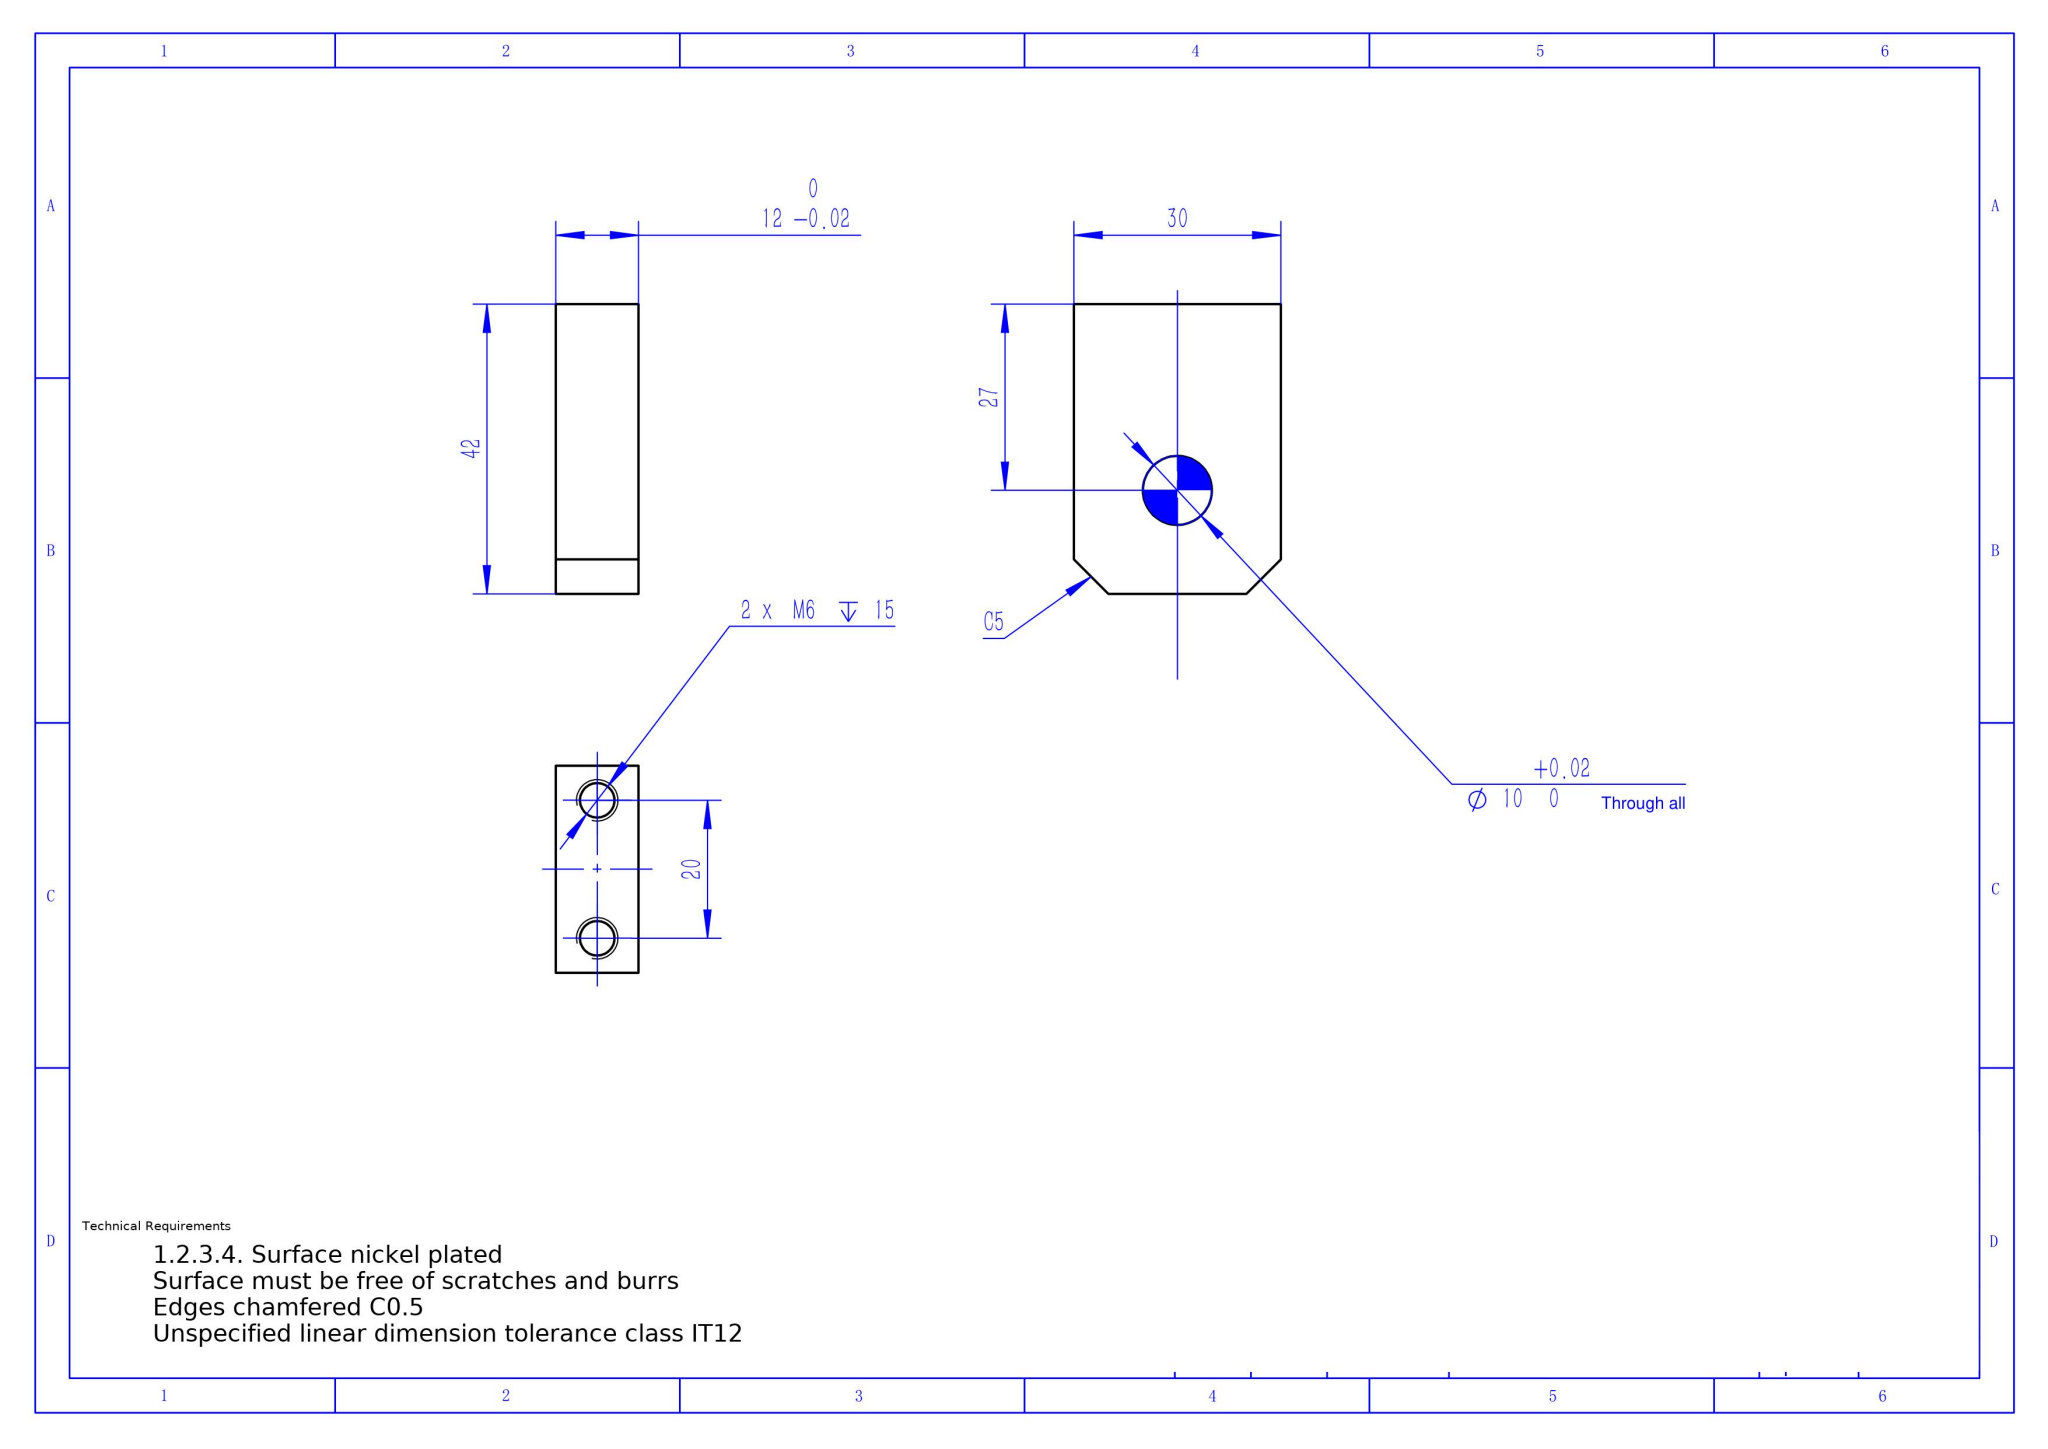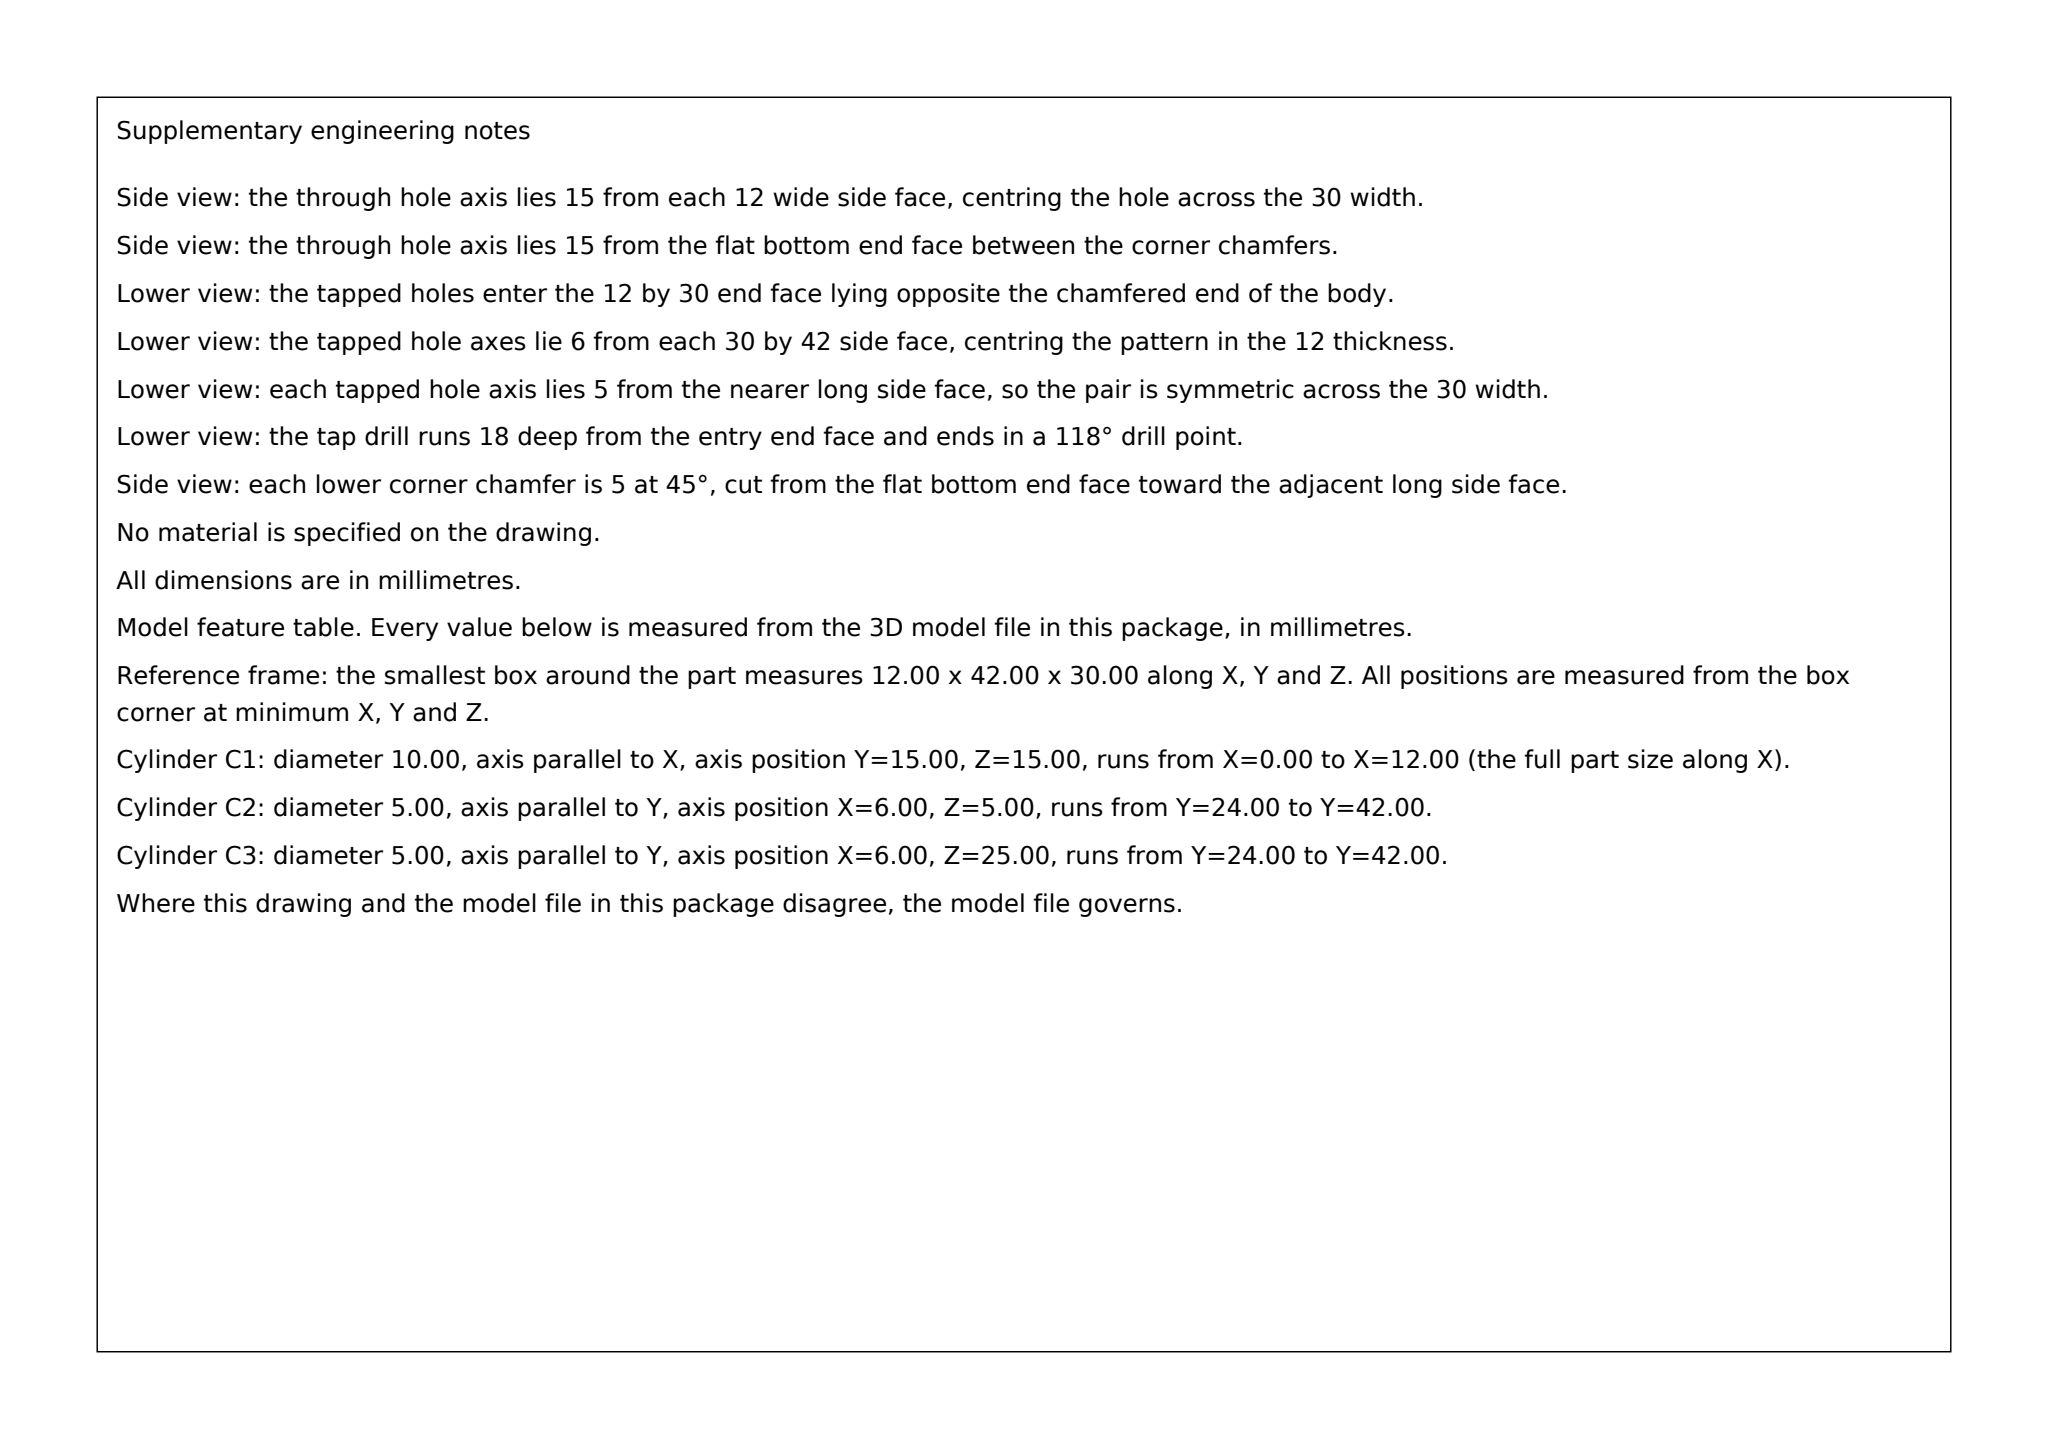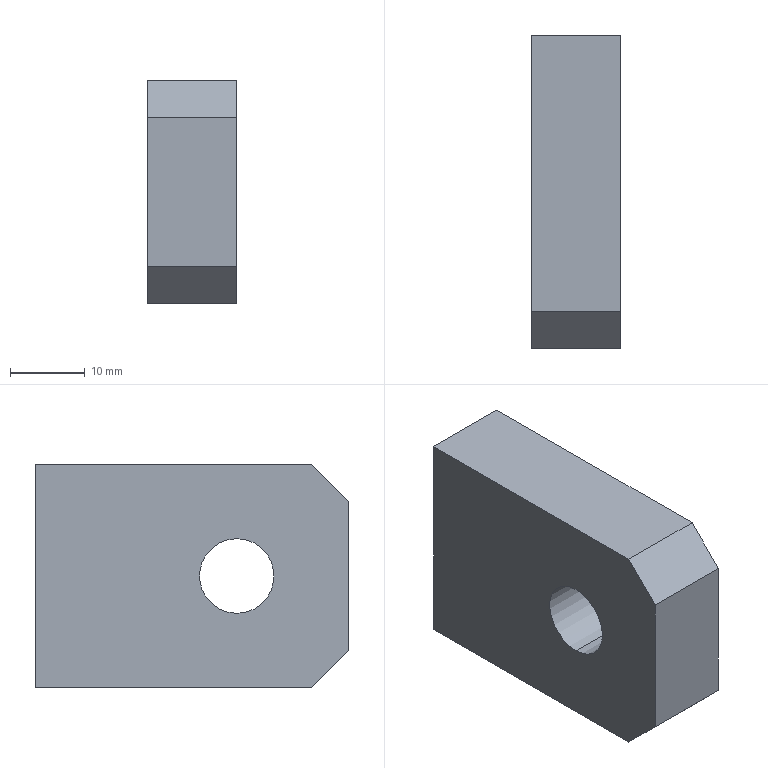Part | SolidWorks | mm | 1 solid | 18 faces | box 12 x 42 x 30 mm | volume 13151 mm3 | plane 8 | cylinder 6 | cone 4 | commonest cylinder face diameters 5 x4 10 x2
build123d program:
from build123d import *

# Parameters (mm, degrees)
SKETCH1_W                  = 30
SKETCH1_H                  = 42
BOSS_EXTRUDE1_DEPTH        = 6
SIZE_MM_DOWEL_PIN_HOLE_1_D = 10
M6_TAPPED_HOLE1_D          = 5
M6_TAPPED_HOLE1_DEPTH      = 18
M6_TAPPED_HOLE1_TIP        = 1.502
CHAMFER1_SIZE              = 5


with BuildPart() as part:
    # Sketch1 → Boss-Extrude1 (new, symmetric)
    with BuildSketch(Plane(origin=(0, 0, 0), x_dir=(0, 0, -1), z_dir=(1, 0, 0))):
        with Locations((0, 21)):
            Rectangle(SKETCH1_W, SKETCH1_H)
    extrude(amount=BOSS_EXTRUDE1_DEPTH, both=True)

    # Size mm Dowel Pin Hole 1 (through all)
    with Locations(Plane(origin=(6, 0, 0), x_dir=(0, 0, -1), z_dir=(1, 0, 0))):
        with Locations((0, 15)):
            Hole(SIZE_MM_DOWEL_PIN_HOLE_1_D / 2)

    # M6 Tapped Hole1
    with Locations(Plane(origin=(0, 42, -226.777), x_dir=(1, 0, 0), z_dir=(0, 1, 0))):
        with Locations((0, -216.777), (0, -236.777)):
            Hole(M6_TAPPED_HOLE1_D / 2, depth=M6_TAPPED_HOLE1_DEPTH)
            with Locations((0, 0, -(M6_TAPPED_HOLE1_DEPTH + M6_TAPPED_HOLE1_TIP / 2))):  # 118° drill point
                Cone(0, M6_TAPPED_HOLE1_D / 2, M6_TAPPED_HOLE1_TIP, mode=Mode.SUBTRACT)

    # Chamfer1
    chamfer1_edges = [part.edges().sort_by_distance(p)[0] for p in [
        (0, 0, -15),
        (0, 0, 15),
    ]]
    chamfer(chamfer1_edges, length=CHAMFER1_SIZE)


solid = part.part
STEP:
#1=CARTESIAN_POINT('',(0.,24.,-12.5));
#2=VERTEX_POINT('',#1);
#3=CARTESIAN_POINT('',(0.,24.,-7.5));
#4=VERTEX_POINT('',#3);
#5=CARTESIAN_POINT('',(0.,24.,-10.));
#6=DIRECTION('',(0.,1.,0.));
#7=DIRECTION('',(0.,0.,1.));
#8=AXIS2_PLACEMENT_3D('',#5,#6,#7);
#9=CIRCLE('',#8,2.5);
#10=EDGE_CURVE('',#2,#4,#9,.T.);
#11=ORIENTED_EDGE('',*,*,#10,.F.);
#12=CARTESIAN_POINT('',(0.,42.,-12.5));
#13=VERTEX_POINT('',#12);
#14=CARTESIAN_POINT('',(0.,42.,-12.5));
#15=DIRECTION('',(0.,1.,0.));
#16=VECTOR('',#15,1000.);
#17=LINE('',#14,#16);
#18=EDGE_CURVE('',#2,#13,#17,.T.);
#19=ORIENTED_EDGE('',*,*,#18,.T.);
#20=CARTESIAN_POINT('',(0.,42.,-7.5));
#21=VERTEX_POINT('',#20);
#22=CARTESIAN_POINT('',(0.,42.,-10.));
#23=DIRECTION('',(0.,1.,0.));
#24=DIRECTION('',(0.,0.,1.));
#25=AXIS2_PLACEMENT_3D('',#22,#23,#24);
#26=CIRCLE('',#25,2.5);
#27=EDGE_CURVE('',#13,#21,#26,.T.);
#28=ORIENTED_EDGE('',*,*,#27,.T.);
#29=CARTESIAN_POINT('',(0.,42.,-7.5));
#30=DIRECTION('',(0.,1.,0.));
#31=VECTOR('',#30,1000.);
#32=LINE('',#29,#31);
#33=EDGE_CURVE('',#4,#21,#32,.T.);
#34=ORIENTED_EDGE('',*,*,#33,.F.);
#35=EDGE_LOOP('',(#11,#19,#28,#34));
#36=FACE_OUTER_BOUND('',#35,.T.);
#37=CARTESIAN_POINT('',(0.,42.,-10.));
#38=DIRECTION('',(0.,1.,0.));
#39=DIRECTION('',(0.,0.,1.));
#40=AXIS2_PLACEMENT_3D('',#37,#38,#39);
#41=CYLINDRICAL_SURFACE('',#40,2.5);
#42=ADVANCED_FACE('',(#36),#41,.F.);
#43=CARTESIAN_POINT('',(-0.,22.498,-10.));
#44=VERTEX_POINT('',#43);
#45=CARTESIAN_POINT('',(0.,24.,-7.5));
#46=DIRECTION('',(0.,0.515,0.8572));
#47=VECTOR('',#46,1000.);
#48=LINE('',#45,#47);
#49=EDGE_CURVE('',#44,#4,#48,.T.);
#50=ORIENTED_EDGE('',*,*,#49,.F.);
#51=CARTESIAN_POINT('',(0.,24.,-12.5));
#52=DIRECTION('',(0.,0.515,-0.8572));
#53=VECTOR('',#52,1000.);
#54=LINE('',#51,#53);
#55=EDGE_CURVE('',#44,#2,#54,.T.);
#56=ORIENTED_EDGE('',*,*,#55,.T.);
#57=ORIENTED_EDGE('',*,*,#10,.T.);
#58=EDGE_LOOP('',(#50,#56,#57));
#59=FACE_OUTER_BOUND('',#58,.T.);
#60=CARTESIAN_POINT('',(0.,24.,-10.));
#61=DIRECTION('',(0.,1.,0.));
#62=DIRECTION('',(0.,0.,1.));
#63=AXIS2_PLACEMENT_3D('',#60,#61,#62);
#64=CONICAL_SURFACE('',#63,2.5,1.03);
#65=ADVANCED_FACE('',(#59),#64,.F.);
#66=CARTESIAN_POINT('',(-0.,24.,7.5));
#67=VERTEX_POINT('',#66);
#68=CARTESIAN_POINT('',(-0.,24.,12.5));
#69=VERTEX_POINT('',#68);
#70=CARTESIAN_POINT('',(-0.,24.,10.));
#71=DIRECTION('',(0.,1.,0.));
#72=DIRECTION('',(0.,0.,1.));
#73=AXIS2_PLACEMENT_3D('',#70,#71,#72);
#74=CIRCLE('',#73,2.5);
#75=EDGE_CURVE('',#67,#69,#74,.T.);
#76=ORIENTED_EDGE('',*,*,#75,.F.);
#77=CARTESIAN_POINT('',(-0.,42.,7.5));
#78=VERTEX_POINT('',#77);
#79=CARTESIAN_POINT('',(-0.,42.,7.5));
#80=DIRECTION('',(0.,1.,0.));
#81=VECTOR('',#80,1000.);
#82=LINE('',#79,#81);
#83=EDGE_CURVE('',#67,#78,#82,.T.);
#84=ORIENTED_EDGE('',*,*,#83,.T.);
#85=CARTESIAN_POINT('',(-0.,42.,12.5));
#86=VERTEX_POINT('',#85);
#87=CARTESIAN_POINT('',(-0.,42.,10.));
#88=DIRECTION('',(0.,1.,0.));
#89=DIRECTION('',(0.,0.,1.));
#90=AXIS2_PLACEMENT_3D('',#87,#88,#89);
#91=CIRCLE('',#90,2.5);
#92=EDGE_CURVE('',#78,#86,#91,.T.);
#93=ORIENTED_EDGE('',*,*,#92,.T.);
#94=CARTESIAN_POINT('',(-0.,42.,12.5));
#95=DIRECTION('',(0.,1.,0.));
#96=VECTOR('',#95,1000.);
#97=LINE('',#94,#96);
#98=EDGE_CURVE('',#69,#86,#97,.T.);
#99=ORIENTED_EDGE('',*,*,#98,.F.);
#100=EDGE_LOOP('',(#76,#84,#93,#99));
#101=FACE_OUTER_BOUND('',#100,.T.);
#102=CARTESIAN_POINT('',(-0.,42.,10.));
#103=DIRECTION('',(0.,1.,0.));
#104=DIRECTION('',(0.,0.,1.));
#105=AXIS2_PLACEMENT_3D('',#102,#103,#104);
#106=CYLINDRICAL_SURFACE('',#105,2.5);
#107=ADVANCED_FACE('',(#101),#106,.F.);
#108=CARTESIAN_POINT('',(-0.,22.498,10.));
#109=VERTEX_POINT('',#108);
#110=CARTESIAN_POINT('',(-0.,24.,12.5));
#111=DIRECTION('',(0.,0.515,0.8572));
#112=VECTOR('',#111,1000.);
#113=LINE('',#110,#112);
#114=EDGE_CURVE('',#109,#69,#113,.T.);
#115=ORIENTED_EDGE('',*,*,#114,.F.);
#116=CARTESIAN_POINT('',(-0.,24.,7.5));
#117=DIRECTION('',(0.,0.515,-0.8572));
#118=VECTOR('',#117,1000.);
#119=LINE('',#116,#118);
#120=EDGE_CURVE('',#109,#67,#119,.T.);
#121=ORIENTED_EDGE('',*,*,#120,.T.);
#122=ORIENTED_EDGE('',*,*,#75,.T.);
#123=EDGE_LOOP('',(#115,#121,#122));
#124=FACE_OUTER_BOUND('',#123,.T.);
#125=CARTESIAN_POINT('',(-0.,24.,10.));
#126=DIRECTION('',(0.,1.,0.));
#127=DIRECTION('',(0.,0.,1.));
#128=AXIS2_PLACEMENT_3D('',#125,#126,#127);
#129=CONICAL_SURFACE('',#128,2.5,1.03);
#130=ADVANCED_FACE('',(#124),#129,.F.);
#131=CARTESIAN_POINT('',(-6.,15.,5.));
#132=VERTEX_POINT('',#131);
#133=CARTESIAN_POINT('',(-6.,15.,-5.));
#134=VERTEX_POINT('',#133);
#135=CARTESIAN_POINT('',(-6.,15.,-0.));
#136=DIRECTION('',(1.,0.,0.));
#137=DIRECTION('',(0.,0.,-1.));
#138=AXIS2_PLACEMENT_3D('',#135,#136,#137);
#139=CIRCLE('',#138,5.);
#140=EDGE_CURVE('',#132,#134,#139,.T.);
#141=ORIENTED_EDGE('',*,*,#140,.F.);
#142=CARTESIAN_POINT('',(6.,15.,5.));
#143=VERTEX_POINT('',#142);
#144=CARTESIAN_POINT('',(6.,15.,5.));
#145=DIRECTION('',(1.,0.,0.));
#146=VECTOR('',#145,1000.);
#147=LINE('',#144,#146);
#148=EDGE_CURVE('',#132,#143,#147,.T.);
#149=ORIENTED_EDGE('',*,*,#148,.T.);
#150=CARTESIAN_POINT('',(6.,15.,-5.));
#151=VERTEX_POINT('',#150);
#152=CARTESIAN_POINT('',(6.,15.,-0.));
#153=DIRECTION('',(1.,0.,0.));
#154=DIRECTION('',(0.,0.,-1.));
#155=AXIS2_PLACEMENT_3D('',#152,#153,#154);
#156=CIRCLE('',#155,5.);
#157=EDGE_CURVE('',#143,#151,#156,.T.);
#158=ORIENTED_EDGE('',*,*,#157,.T.);
#159=CARTESIAN_POINT('',(6.,15.,-5.));
#160=DIRECTION('',(1.,0.,0.));
#161=VECTOR('',#160,1000.);
#162=LINE('',#159,#161);
#163=EDGE_CURVE('',#134,#151,#162,.T.);
#164=ORIENTED_EDGE('',*,*,#163,.F.);
#165=EDGE_LOOP('',(#141,#149,#158,#164));
#166=FACE_OUTER_BOUND('',#165,.T.);
#167=CARTESIAN_POINT('',(6.,15.,-0.));
#168=DIRECTION('',(1.,0.,0.));
#169=DIRECTION('',(0.,0.,-1.));
#170=AXIS2_PLACEMENT_3D('',#167,#168,#169);
#171=CYLINDRICAL_SURFACE('',#170,5.);
#172=ADVANCED_FACE('',(#166),#171,.F.);
#173=CARTESIAN_POINT('',(-6.,42.,15.));
#174=VERTEX_POINT('',#173);
#175=CARTESIAN_POINT('',(-6.,5.,15.));
#176=VERTEX_POINT('',#175);
#177=CARTESIAN_POINT('',(-6.,0.,15.));
#178=DIRECTION('',(0.,-1.,0.));
#179=VECTOR('',#178,1000.);
#180=LINE('',#177,#179);
#181=EDGE_CURVE('',#174,#176,#180,.T.);
#182=ORIENTED_EDGE('',*,*,#181,.T.);
#183=CARTESIAN_POINT('',(6.,5.,15.));
#184=VERTEX_POINT('',#183);
#185=CARTESIAN_POINT('',(6.,5.,15.));
#186=DIRECTION('',(1.,0.,0.));
#187=VECTOR('',#186,1000.);
#188=LINE('',#185,#187);
#189=EDGE_CURVE('',#176,#184,#188,.T.);
#190=ORIENTED_EDGE('',*,*,#189,.T.);
#191=CARTESIAN_POINT('',(6.,42.,15.));
#192=VERTEX_POINT('',#191);
#193=CARTESIAN_POINT('',(6.,0.,15.));
#194=DIRECTION('',(0.,-1.,0.));
#195=VECTOR('',#194,1000.);
#196=LINE('',#193,#195);
#197=EDGE_CURVE('',#192,#184,#196,.T.);
#198=ORIENTED_EDGE('',*,*,#197,.F.);
#199=CARTESIAN_POINT('',(6.,42.,15.));
#200=DIRECTION('',(-1.,0.,0.));
#201=VECTOR('',#200,1000.);
#202=LINE('',#199,#201);
#203=EDGE_CURVE('',#192,#174,#202,.T.);
#204=ORIENTED_EDGE('',*,*,#203,.T.);
#205=EDGE_LOOP('',(#182,#190,#198,#204));
#206=FACE_OUTER_BOUND('',#205,.T.);
#207=CARTESIAN_POINT('',(6.,0.,15.));
#208=DIRECTION('',(0.,0.,-1.));
#209=DIRECTION('',(-1.,0.,0.));
#210=AXIS2_PLACEMENT_3D('',#207,#208,#209);
#211=PLANE('',#210);
#212=ADVANCED_FACE('',(#206),#211,.F.);
#213=CARTESIAN_POINT('',(-6.,0.,10.));
#214=VERTEX_POINT('',#213);
#215=CARTESIAN_POINT('',(-6.,0.,-10.));
#216=VERTEX_POINT('',#215);
#217=CARTESIAN_POINT('',(-6.,0.,15.));
#218=DIRECTION('',(0.,0.,-1.));
#219=VECTOR('',#218,1000.);
#220=LINE('',#217,#219);
#221=EDGE_CURVE('',#214,#216,#220,.T.);
#222=ORIENTED_EDGE('',*,*,#221,.T.);
#223=CARTESIAN_POINT('',(6.,0.,-10.));
#224=VERTEX_POINT('',#223);
#225=CARTESIAN_POINT('',(6.,0.,-10.));
#226=DIRECTION('',(1.,0.,0.));
#227=VECTOR('',#226,1000.);
#228=LINE('',#225,#227);
#229=EDGE_CURVE('',#216,#224,#228,.T.);
#230=ORIENTED_EDGE('',*,*,#229,.T.);
#231=CARTESIAN_POINT('',(6.,0.,10.));
#232=VERTEX_POINT('',#231);
#233=CARTESIAN_POINT('',(6.,0.,15.));
#234=DIRECTION('',(0.,0.,-1.));
#235=VECTOR('',#234,1000.);
#236=LINE('',#233,#235);
#237=EDGE_CURVE('',#232,#224,#236,.T.);
#238=ORIENTED_EDGE('',*,*,#237,.F.);
#239=CARTESIAN_POINT('',(6.,0.,10.));
#240=DIRECTION('',(-1.,0.,0.));
#241=VECTOR('',#240,1000.);
#242=LINE('',#239,#241);
#243=EDGE_CURVE('',#232,#214,#242,.T.);
#244=ORIENTED_EDGE('',*,*,#243,.T.);
#245=EDGE_LOOP('',(#222,#230,#238,#244));
#246=FACE_OUTER_BOUND('',#245,.T.);
#247=CARTESIAN_POINT('',(6.,0.,15.));
#248=DIRECTION('',(0.,1.,0.));
#249=DIRECTION('',(0.,0.,1.));
#250=AXIS2_PLACEMENT_3D('',#247,#248,#249);
#251=PLANE('',#250);
#252=ADVANCED_FACE('',(#246),#251,.F.);
#253=CARTESIAN_POINT('',(6.,5.,-15.));
#254=VERTEX_POINT('',#253);
#255=CARTESIAN_POINT('',(6.,42.,-15.));
#256=VERTEX_POINT('',#255);
#257=CARTESIAN_POINT('',(6.,0.,-15.));
#258=DIRECTION('',(0.,1.,0.));
#259=VECTOR('',#258,1000.);
#260=LINE('',#257,#259);
#261=EDGE_CURVE('',#254,#256,#260,.T.);
#262=ORIENTED_EDGE('',*,*,#261,.F.);
#263=CARTESIAN_POINT('',(-6.,5.,-15.));
#264=VERTEX_POINT('',#263);
#265=CARTESIAN_POINT('',(6.,5.,-15.));
#266=DIRECTION('',(-1.,0.,0.));
#267=VECTOR('',#266,1000.);
#268=LINE('',#265,#267);
#269=EDGE_CURVE('',#254,#264,#268,.T.);
#270=ORIENTED_EDGE('',*,*,#269,.T.);
#271=CARTESIAN_POINT('',(-6.,42.,-15.));
#272=VERTEX_POINT('',#271);
#273=CARTESIAN_POINT('',(-6.,0.,-15.));
#274=DIRECTION('',(0.,1.,0.));
#275=VECTOR('',#274,1000.);
#276=LINE('',#273,#275);
#277=EDGE_CURVE('',#264,#272,#276,.T.);
#278=ORIENTED_EDGE('',*,*,#277,.T.);
#279=CARTESIAN_POINT('',(6.,42.,-15.));
#280=DIRECTION('',(-1.,0.,0.));
#281=VECTOR('',#280,1000.);
#282=LINE('',#279,#281);
#283=EDGE_CURVE('',#256,#272,#282,.T.);
#284=ORIENTED_EDGE('',*,*,#283,.F.);
#285=EDGE_LOOP('',(#262,#270,#278,#284));
#286=FACE_OUTER_BOUND('',#285,.T.);
#287=CARTESIAN_POINT('',(6.,0.,-15.));
#288=DIRECTION('',(0.,0.,1.));
#289=DIRECTION('',(1.,0.,0.));
#290=AXIS2_PLACEMENT_3D('',#287,#288,#289);
#291=PLANE('',#290);
#292=ADVANCED_FACE('',(#286),#291,.F.);
#293=CARTESIAN_POINT('',(0.,42.,-10.));
#294=DIRECTION('',(0.,1.,0.));
#295=DIRECTION('',(0.,0.,1.));
#296=AXIS2_PLACEMENT_3D('',#293,#294,#295);
#297=CIRCLE('',#296,2.5);
#298=EDGE_CURVE('',#21,#13,#297,.T.);
#299=ORIENTED_EDGE('',*,*,#298,.F.);
#300=ORIENTED_EDGE('',*,*,#27,.F.);
#301=EDGE_LOOP('',(#299,#300));
#302=FACE_BOUND('',#301,.T.);
#303=CARTESIAN_POINT('',(-0.,42.,10.));
#304=DIRECTION('',(0.,1.,0.));
#305=DIRECTION('',(0.,0.,1.));
#306=AXIS2_PLACEMENT_3D('',#303,#304,#305);
#307=CIRCLE('',#306,2.5);
#308=EDGE_CURVE('',#86,#78,#307,.T.);
#309=ORIENTED_EDGE('',*,*,#308,.F.);
#310=ORIENTED_EDGE('',*,*,#92,.F.);
#311=EDGE_LOOP('',(#309,#310));
#312=FACE_BOUND('',#311,.T.);
#313=CARTESIAN_POINT('',(-6.,42.,15.));
#314=DIRECTION('',(0.,0.,1.));
#315=VECTOR('',#314,1000.);
#316=LINE('',#313,#315);
#317=EDGE_CURVE('',#272,#174,#316,.T.);
#318=ORIENTED_EDGE('',*,*,#317,.T.);
#319=ORIENTED_EDGE('',*,*,#203,.F.);
#320=CARTESIAN_POINT('',(6.,42.,15.));
#321=DIRECTION('',(0.,0.,1.));
#322=VECTOR('',#321,1000.);
#323=LINE('',#320,#322);
#324=EDGE_CURVE('',#256,#192,#323,.T.);
#325=ORIENTED_EDGE('',*,*,#324,.F.);
#326=ORIENTED_EDGE('',*,*,#283,.T.);
#327=EDGE_LOOP('',(#318,#319,#325,#326));
#328=FACE_OUTER_BOUND('',#327,.T.);
#329=CARTESIAN_POINT('',(6.,42.,15.));
#330=DIRECTION('',(0.,-1.,0.));
#331=DIRECTION('',(0.,0.,-1.));
#332=AXIS2_PLACEMENT_3D('',#329,#330,#331);
#333=PLANE('',#332);
#334=ADVANCED_FACE('',(#302,#312,#328),#333,.F.);
#335=CARTESIAN_POINT('',(6.,15.,-0.));
#336=DIRECTION('',(1.,0.,0.));
#337=DIRECTION('',(0.,0.,-1.));
#338=AXIS2_PLACEMENT_3D('',#335,#336,#337);
#339=CIRCLE('',#338,5.);
#340=EDGE_CURVE('',#151,#143,#339,.T.);
#341=ORIENTED_EDGE('',*,*,#340,.F.);
#342=ORIENTED_EDGE('',*,*,#157,.F.);
#343=EDGE_LOOP('',(#341,#342));
#344=FACE_BOUND('',#343,.T.);
#345=ORIENTED_EDGE('',*,*,#237,.T.);
#346=CARTESIAN_POINT('',(6.,5.,-15.));
#347=DIRECTION('',(0.,0.7071,-0.7071));
#348=VECTOR('',#347,1000.);
#349=LINE('',#346,#348);
#350=EDGE_CURVE('',#224,#254,#349,.T.);
#351=ORIENTED_EDGE('',*,*,#350,.T.);
#352=ORIENTED_EDGE('',*,*,#261,.T.);
#353=ORIENTED_EDGE('',*,*,#324,.T.);
#354=ORIENTED_EDGE('',*,*,#197,.T.);
#355=CARTESIAN_POINT('',(6.,0.,10.));
#356=DIRECTION('',(0.,-0.7071,-0.7071));
#357=VECTOR('',#356,1000.);
#358=LINE('',#355,#357);
#359=EDGE_CURVE('',#184,#232,#358,.T.);
#360=ORIENTED_EDGE('',*,*,#359,.T.);
#361=EDGE_LOOP('',(#345,#351,#352,#353,#354,#360));
#362=FACE_OUTER_BOUND('',#361,.T.);
#363=CARTESIAN_POINT('',(6.,0.,0.));
#364=DIRECTION('',(-1.,0.,0.));
#365=DIRECTION('',(0.,0.,1.));
#366=AXIS2_PLACEMENT_3D('',#363,#364,#365);
#367=PLANE('',#366);
#368=ADVANCED_FACE('',(#344,#362),#367,.F.);
#369=CARTESIAN_POINT('',(-6.,15.,-0.));
#370=DIRECTION('',(1.,0.,0.));
#371=DIRECTION('',(0.,0.,-1.));
#372=AXIS2_PLACEMENT_3D('',#369,#370,#371);
#373=CIRCLE('',#372,5.);
#374=EDGE_CURVE('',#134,#132,#373,.T.);
#375=ORIENTED_EDGE('',*,*,#374,.T.);
#376=ORIENTED_EDGE('',*,*,#140,.T.);
#377=EDGE_LOOP('',(#375,#376));
#378=FACE_BOUND('',#377,.T.);
#379=ORIENTED_EDGE('',*,*,#277,.F.);
#380=CARTESIAN_POINT('',(-6.,-5.,-5.));
#381=DIRECTION('',(0.,-0.7071,0.7071));
#382=VECTOR('',#381,1000.);
#383=LINE('',#380,#382);
#384=EDGE_CURVE('',#264,#216,#383,.T.);
#385=ORIENTED_EDGE('',*,*,#384,.T.);
#386=ORIENTED_EDGE('',*,*,#221,.F.);
#387=CARTESIAN_POINT('',(-6.,-5.,5.));
#388=DIRECTION('',(0.,0.7071,0.7071));
#389=VECTOR('',#388,1000.);
#390=LINE('',#387,#389);
#391=EDGE_CURVE('',#214,#176,#390,.T.);
#392=ORIENTED_EDGE('',*,*,#391,.T.);
#393=ORIENTED_EDGE('',*,*,#181,.F.);
#394=ORIENTED_EDGE('',*,*,#317,.F.);
#395=EDGE_LOOP('',(#379,#385,#386,#392,#393,#394));
#396=FACE_OUTER_BOUND('',#395,.T.);
#397=CARTESIAN_POINT('',(-6.,0.,0.));
#398=DIRECTION('',(-1.,0.,0.));
#399=DIRECTION('',(0.,0.,1.));
#400=AXIS2_PLACEMENT_3D('',#397,#398,#399);
#401=PLANE('',#400);
#402=ADVANCED_FACE('',(#378,#396),#401,.T.);
#403=ORIENTED_EDGE('',*,*,#148,.F.);
#404=ORIENTED_EDGE('',*,*,#374,.F.);
#405=ORIENTED_EDGE('',*,*,#163,.T.);
#406=ORIENTED_EDGE('',*,*,#340,.T.);
#407=EDGE_LOOP('',(#403,#404,#405,#406));
#408=FACE_OUTER_BOUND('',#407,.T.);
#409=CARTESIAN_POINT('',(6.,15.,-0.));
#410=DIRECTION('',(1.,0.,0.));
#411=DIRECTION('',(0.,0.,-1.));
#412=AXIS2_PLACEMENT_3D('',#409,#410,#411);
#413=CYLINDRICAL_SURFACE('',#412,5.);
#414=ADVANCED_FACE('',(#408),#413,.F.);
#415=ORIENTED_EDGE('',*,*,#120,.F.);
#416=ORIENTED_EDGE('',*,*,#114,.T.);
#417=CARTESIAN_POINT('',(-0.,24.,10.));
#418=DIRECTION('',(0.,1.,0.));
#419=DIRECTION('',(0.,0.,1.));
#420=AXIS2_PLACEMENT_3D('',#417,#418,#419);
#421=CIRCLE('',#420,2.5);
#422=EDGE_CURVE('',#69,#67,#421,.T.);
#423=ORIENTED_EDGE('',*,*,#422,.T.);
#424=EDGE_LOOP('',(#415,#416,#423));
#425=FACE_OUTER_BOUND('',#424,.T.);
#426=CARTESIAN_POINT('',(-0.,24.,10.));
#427=DIRECTION('',(0.,1.,0.));
#428=DIRECTION('',(0.,0.,1.));
#429=AXIS2_PLACEMENT_3D('',#426,#427,#428);
#430=CONICAL_SURFACE('',#429,2.5,1.03);
#431=ADVANCED_FACE('',(#425),#430,.F.);
#432=ORIENTED_EDGE('',*,*,#83,.F.);
#433=ORIENTED_EDGE('',*,*,#422,.F.);
#434=ORIENTED_EDGE('',*,*,#98,.T.);
#435=ORIENTED_EDGE('',*,*,#308,.T.);
#436=EDGE_LOOP('',(#432,#433,#434,#435));
#437=FACE_OUTER_BOUND('',#436,.T.);
#438=CARTESIAN_POINT('',(-0.,42.,10.));
#439=DIRECTION('',(0.,1.,0.));
#440=DIRECTION('',(0.,0.,1.));
#441=AXIS2_PLACEMENT_3D('',#438,#439,#440);
#442=CYLINDRICAL_SURFACE('',#441,2.5);
#443=ADVANCED_FACE('',(#437),#442,.F.);
#444=ORIENTED_EDGE('',*,*,#55,.F.);
#445=ORIENTED_EDGE('',*,*,#49,.T.);
#446=CARTESIAN_POINT('',(0.,24.,-10.));
#447=DIRECTION('',(0.,1.,0.));
#448=DIRECTION('',(0.,0.,1.));
#449=AXIS2_PLACEMENT_3D('',#446,#447,#448);
#450=CIRCLE('',#449,2.5);
#451=EDGE_CURVE('',#4,#2,#450,.T.);
#452=ORIENTED_EDGE('',*,*,#451,.T.);
#453=EDGE_LOOP('',(#444,#445,#452));
#454=FACE_OUTER_BOUND('',#453,.T.);
#455=CARTESIAN_POINT('',(0.,24.,-10.));
#456=DIRECTION('',(0.,1.,0.));
#457=DIRECTION('',(0.,0.,1.));
#458=AXIS2_PLACEMENT_3D('',#455,#456,#457);
#459=CONICAL_SURFACE('',#458,2.5,1.03);
#460=ADVANCED_FACE('',(#454),#459,.F.);
#461=ORIENTED_EDGE('',*,*,#18,.F.);
#462=ORIENTED_EDGE('',*,*,#451,.F.);
#463=ORIENTED_EDGE('',*,*,#33,.T.);
#464=ORIENTED_EDGE('',*,*,#298,.T.);
#465=EDGE_LOOP('',(#461,#462,#463,#464));
#466=FACE_OUTER_BOUND('',#465,.T.);
#467=CARTESIAN_POINT('',(0.,42.,-10.));
#468=DIRECTION('',(0.,1.,0.));
#469=DIRECTION('',(0.,0.,1.));
#470=AXIS2_PLACEMENT_3D('',#467,#468,#469);
#471=CYLINDRICAL_SURFACE('',#470,2.5);
#472=ADVANCED_FACE('',(#466),#471,.F.);
#473=ORIENTED_EDGE('',*,*,#350,.F.);
#474=ORIENTED_EDGE('',*,*,#229,.F.);
#475=ORIENTED_EDGE('',*,*,#384,.F.);
#476=ORIENTED_EDGE('',*,*,#269,.F.);
#477=EDGE_LOOP('',(#473,#474,#475,#476));
#478=FACE_OUTER_BOUND('',#477,.T.);
#479=CARTESIAN_POINT('',(6.,5.,-15.));
#480=DIRECTION('',(0.,0.7071,0.7071));
#481=DIRECTION('',(-1.,0.,0.));
#482=AXIS2_PLACEMENT_3D('',#479,#480,#481);
#483=PLANE('',#482);
#484=ADVANCED_FACE('',(#478),#483,.F.);
#485=ORIENTED_EDGE('',*,*,#359,.F.);
#486=ORIENTED_EDGE('',*,*,#189,.F.);
#487=ORIENTED_EDGE('',*,*,#391,.F.);
#488=ORIENTED_EDGE('',*,*,#243,.F.);
#489=EDGE_LOOP('',(#485,#486,#487,#488));
#490=FACE_OUTER_BOUND('',#489,.T.);
#491=CARTESIAN_POINT('',(6.,0.,10.));
#492=DIRECTION('',(0.,0.7071,-0.7071));
#493=DIRECTION('',(-1.,0.,0.));
#494=AXIS2_PLACEMENT_3D('',#491,#492,#493);
#495=PLANE('',#494);
#496=ADVANCED_FACE('',(#490),#495,.F.);
#497=CLOSED_SHELL('',(#42,#65,#107,#130,#172,#212,#252,#292,#334,#368,#402,#414,#431,#443,#460,#472,#484,#496));
#498=MANIFOLD_SOLID_BREP('',#497);
#499=CARTESIAN_POINT('',(0.,0.,0.));
#500=DIRECTION('',(0.,0.,1.));
#501=DIRECTION('',(1.,0.,0.));
#502=AXIS2_PLACEMENT_3D('',#499,#500,#501);
#503=(LENGTH_UNIT()NAMED_UNIT(*)SI_UNIT(.MILLI.,.METRE.));
#504=UNCERTAINTY_MEASURE_WITH_UNIT(LENGTH_MEASURE(0.00001),#503,'','');
#505=(NAMED_UNIT(*)PLANE_ANGLE_UNIT()SI_UNIT($,.RADIAN.));
#506=(NAMED_UNIT(*)SI_UNIT($,.STERADIAN.)SOLID_ANGLE_UNIT());
#507=(GEOMETRIC_REPRESENTATION_CONTEXT(3)GLOBAL_UNCERTAINTY_ASSIGNED_CONTEXT((#504))GLOBAL_UNIT_ASSIGNED_CONTEXT((#503,#505,#506))REPRESENTATION_CONTEXT('',''));
#508=ADVANCED_BREP_SHAPE_REPRESENTATION('',(#498,#502),#507);